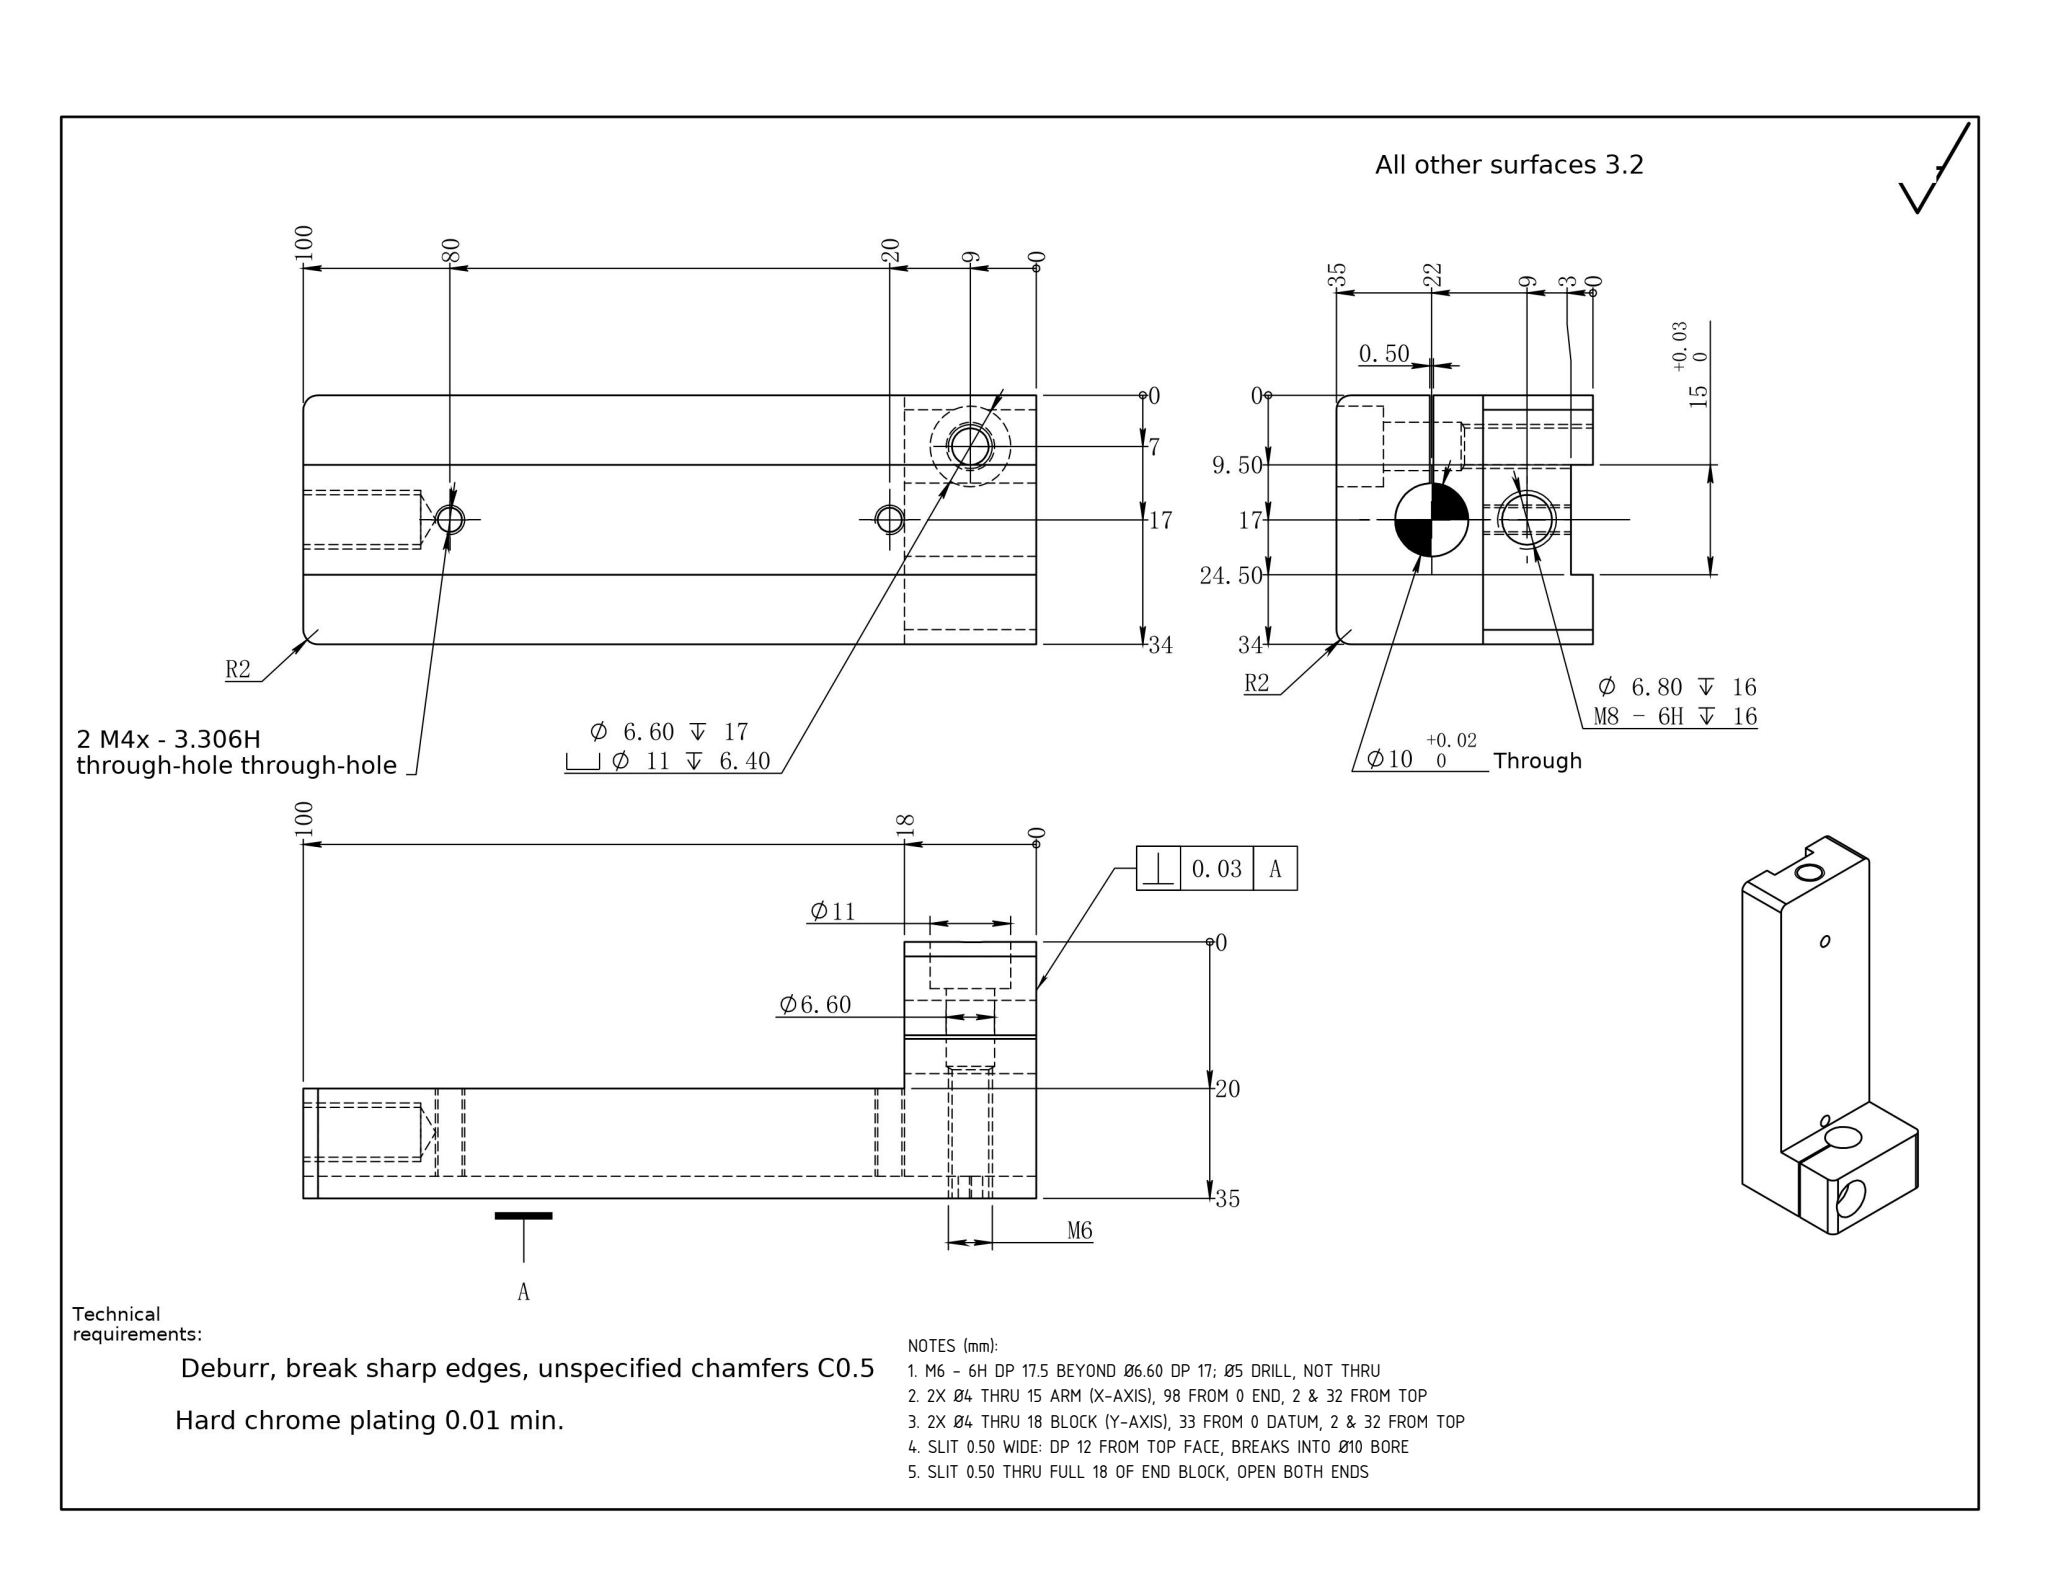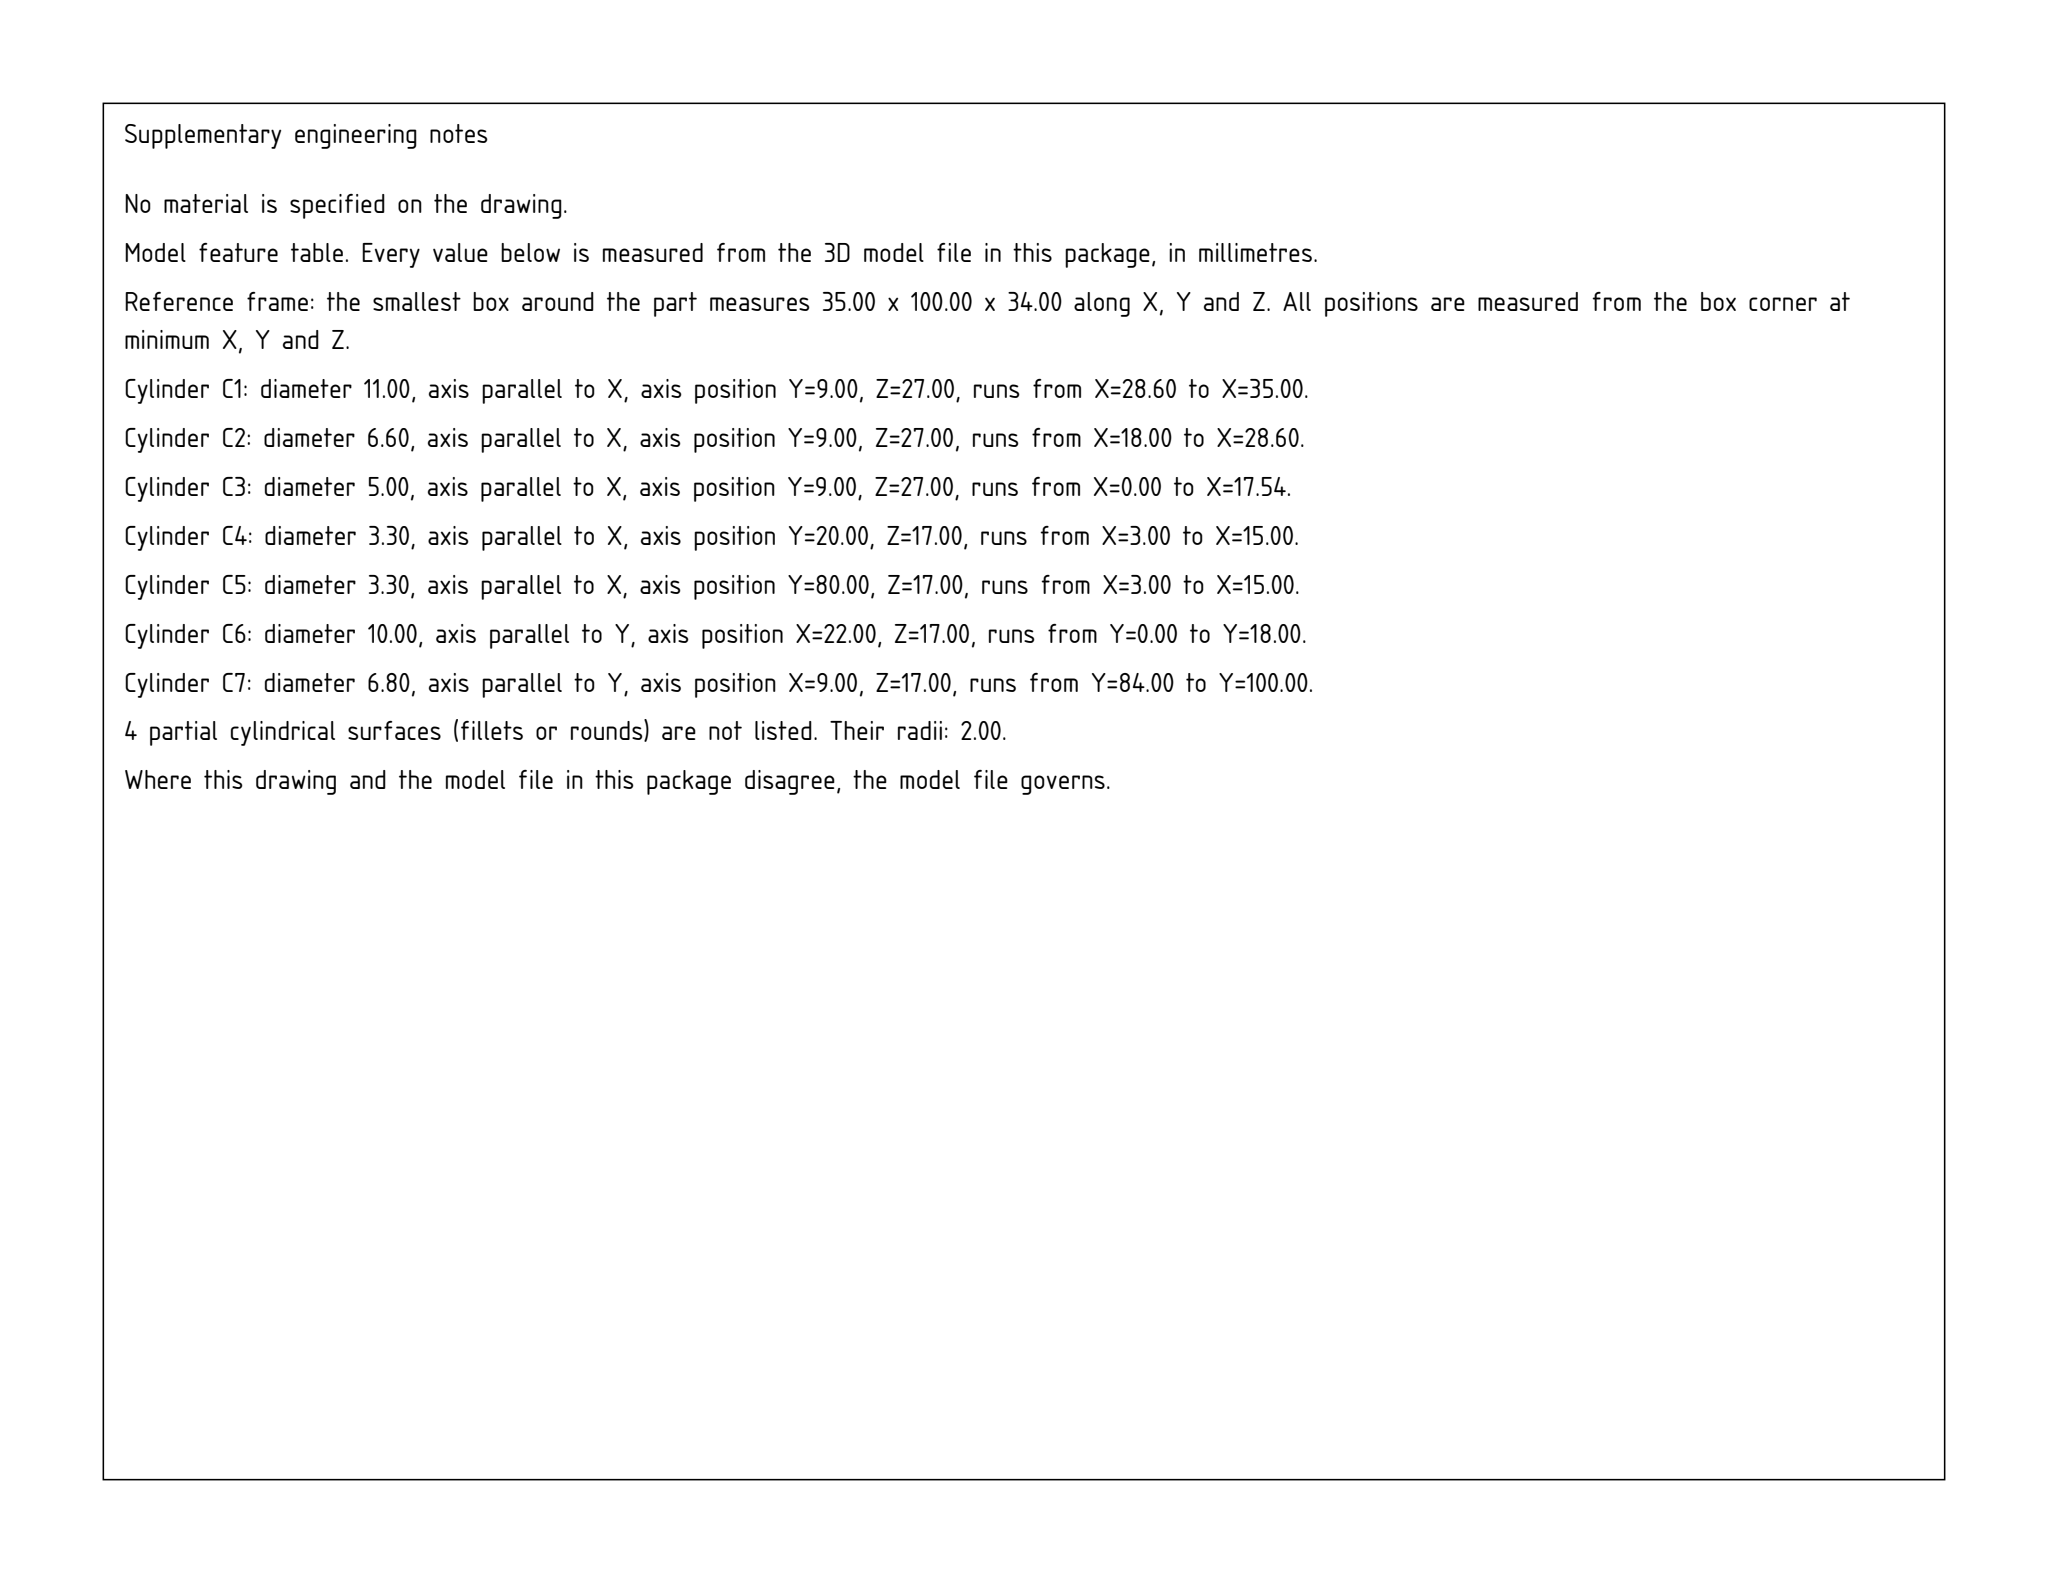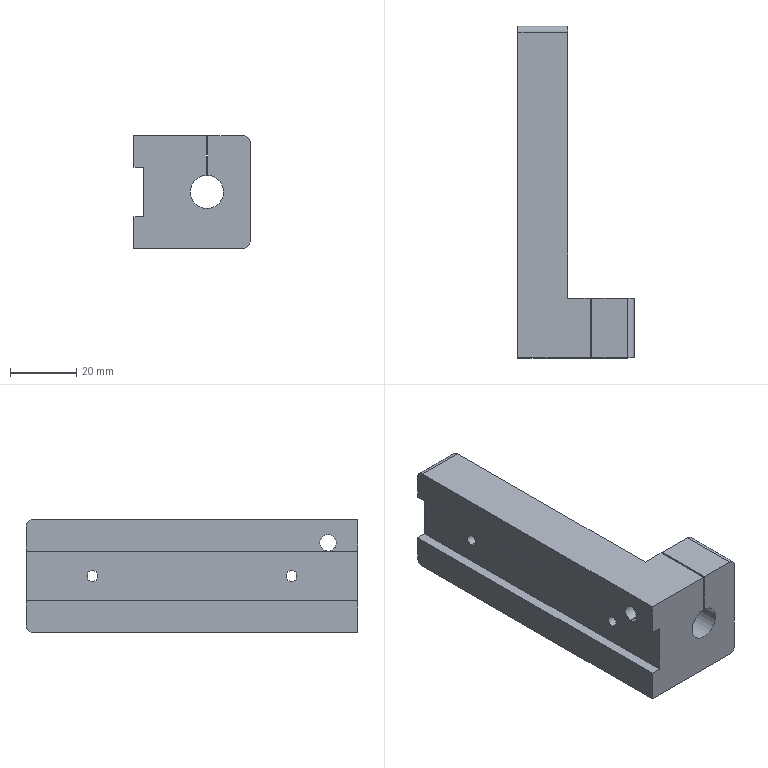Part | SolidWorks | mm | 1 solid | 42 faces | box 35 x 100 x 34 mm | volume 55040 mm3 | cylinder 21 | plane 17 | cone 4 | commonest cylinder face diameters 3.3 x4 6.6 x4 4 x4 10 x3 6.8 x2 11 x2 5 x2
Drawing notes:
M6 - 6H DP 17.5 BEYOND Ø6.60 DP 17; Ø5 DRILL, NOT THRU | from the solid: Ø5.0 cyl, axis x, at y=9.0 z=27.0, length 17.54, spanning x=0.46 to x=18.0; coaxial with Ø6.60 (x=18..28.6) and Ø11 ↧6.4 (x=28.6..35) entering the x=35 face
2X Ø4 THRU 15 ARM (X-AXIS), 98 FROM 0 END, 2 & 32 FROM TOP | from the solid: cylinders [4.0,"x",[null,98.0,2.0],15.0] and [4.0,"x",[null,98.0,32.0],15.0]; bbox Y=100, Z=34
2X Ø4 THRU 18 BLOCK (Y-AXIS), 33 FROM 0 DATUM, 2 & 32 FROM TOP | from the solid: cylinders [4.0,"y",[33.0,null,2.0],18.0] and [4.0,"y",[33.0,null,32.0],18.0]; bbox X=35, Z=34
SLIT 0.50 WIDE: DP 12 FROM TOP FACE, BREAKS INTO Ø10 BORE | from the solid: Slit faces x=21.75/22.25 open at z=34 plane (split into 2 faces); bottom ends on Ø10 bore, axis z=17, so depth = 17-5 = 12 from top face
SLIT 0.50 THRU FULL 18 OF END BLOCK, OPEN BOTH ENDS | from the solid: Slit runs y=0 to y=18 between block faces y=0 and y=18; Ø10 bore y-length 18 split into 3 faces by slit